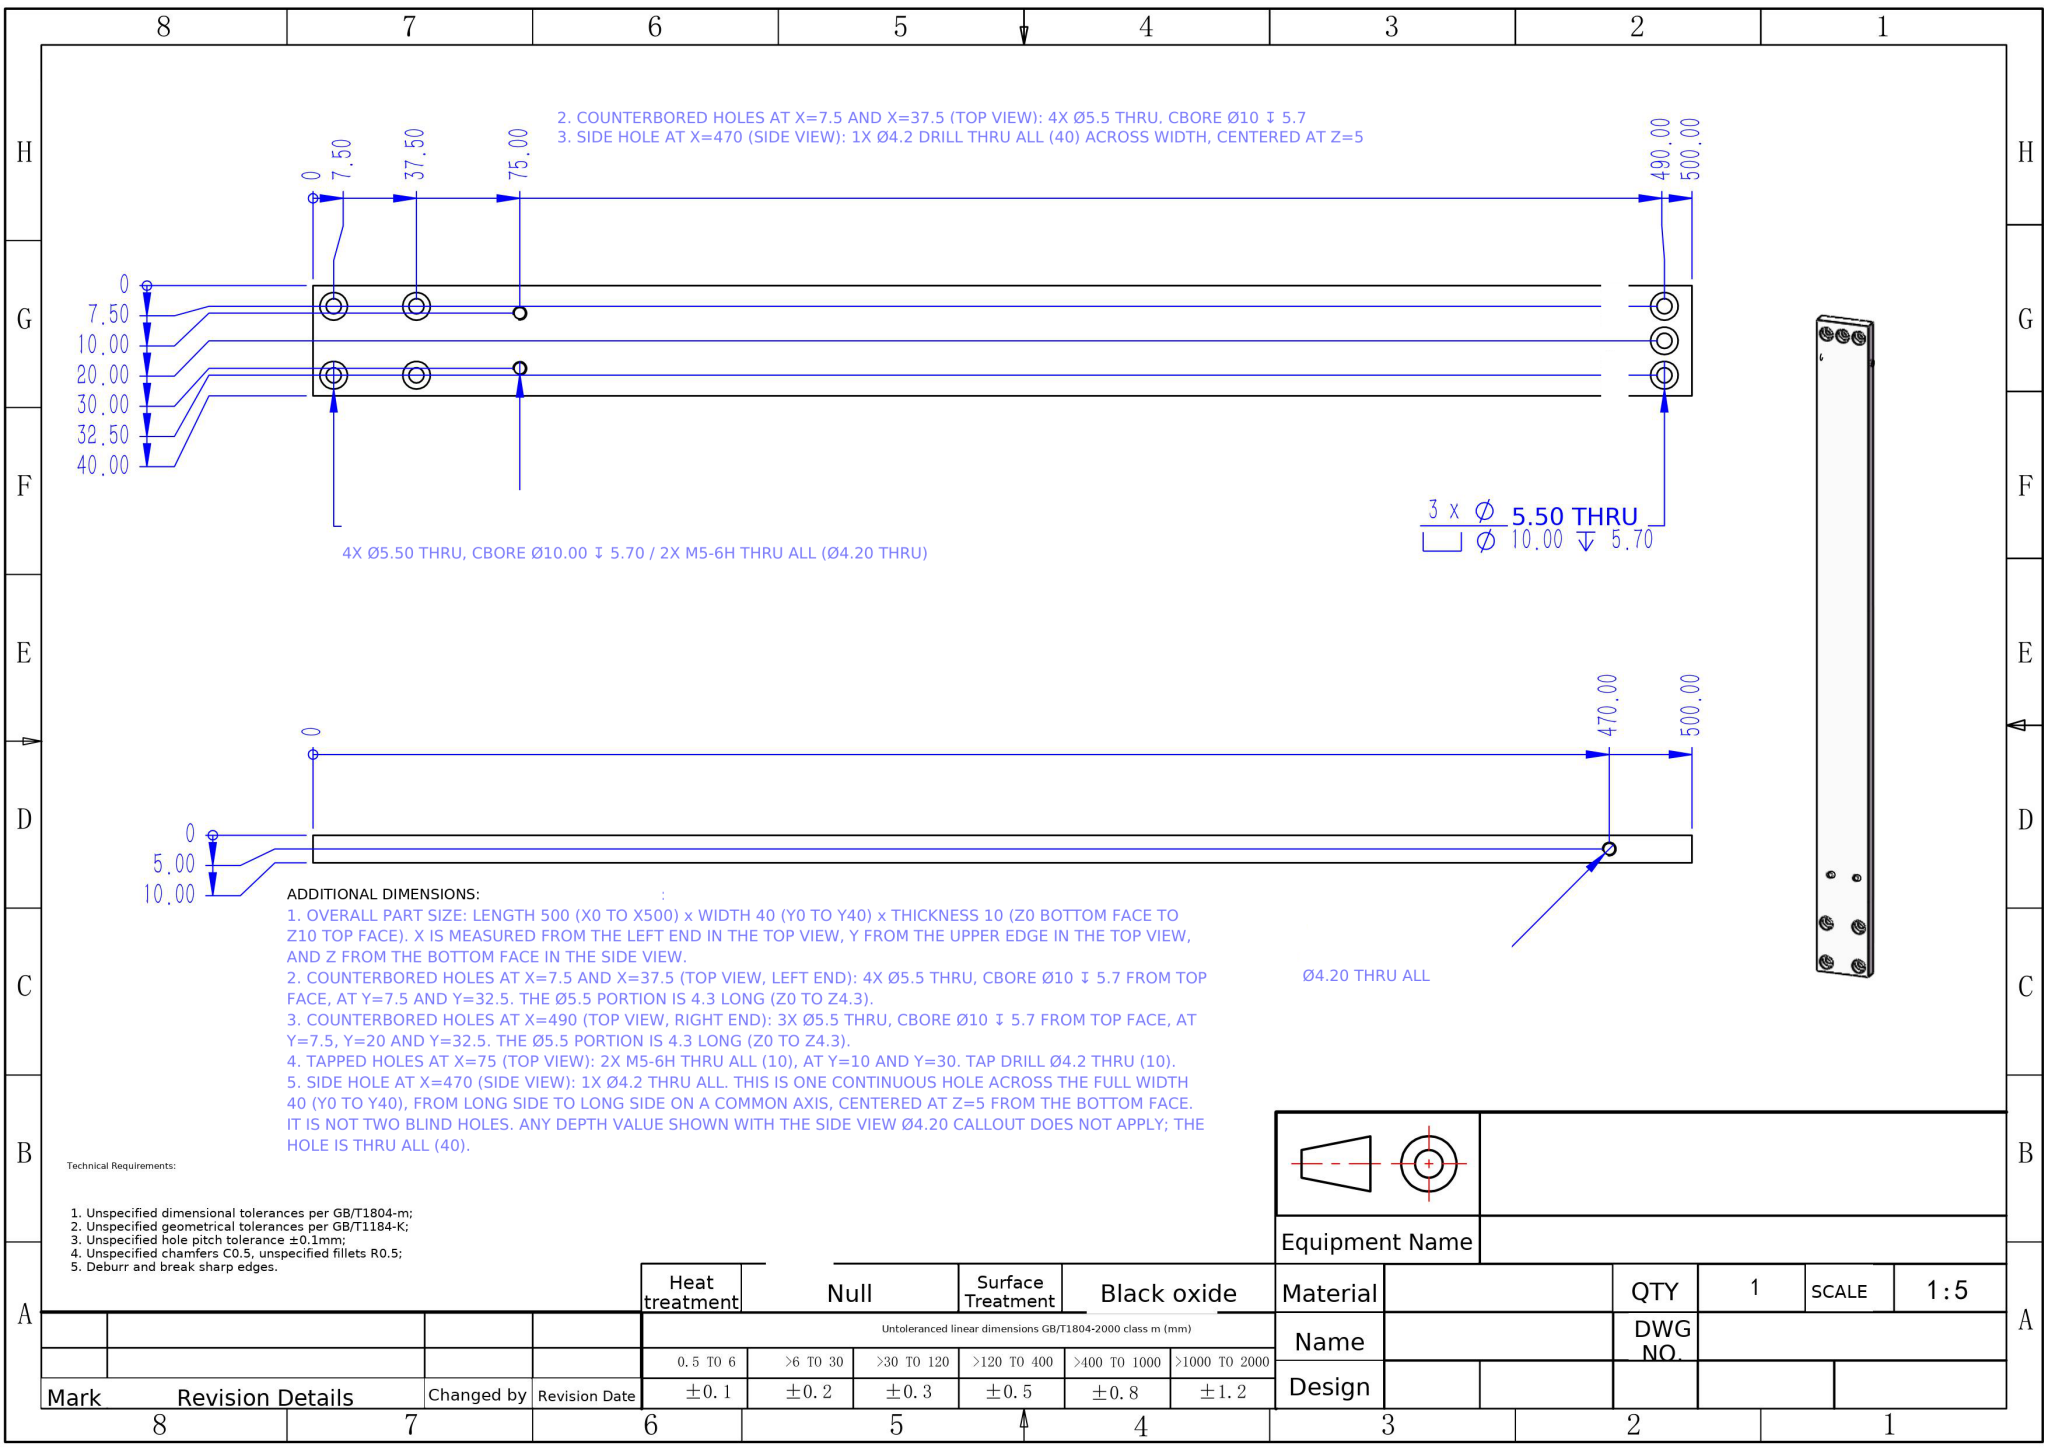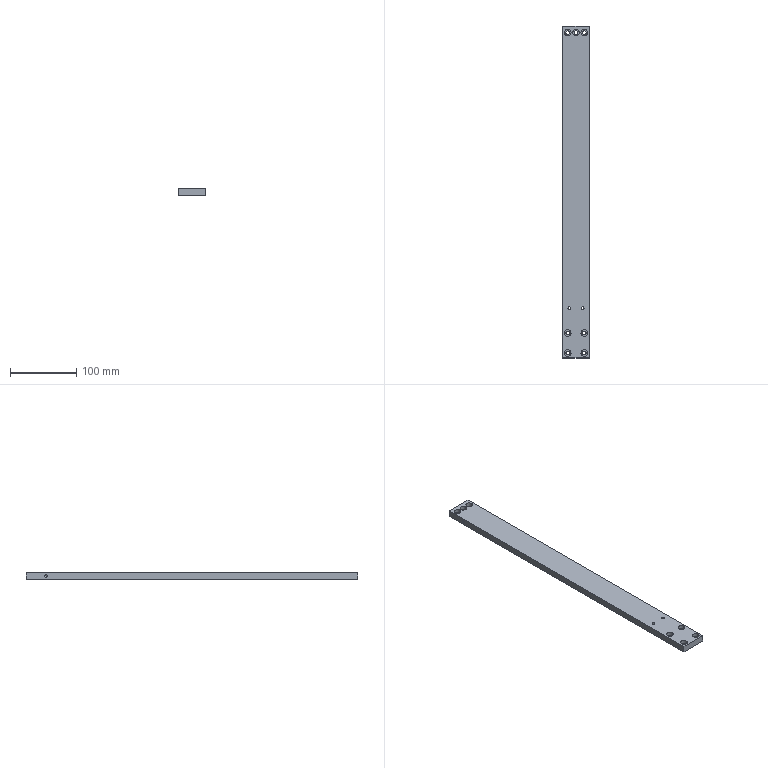Part | NX | mm | 1 solid | 53 faces | box 40 x 500 x 10 mm | volume 195474 mm3 | cylinder 36 | plane 13 | cone 4 | commonest cylinder face diameters 10 x14 5.5 x14 4.2 x8